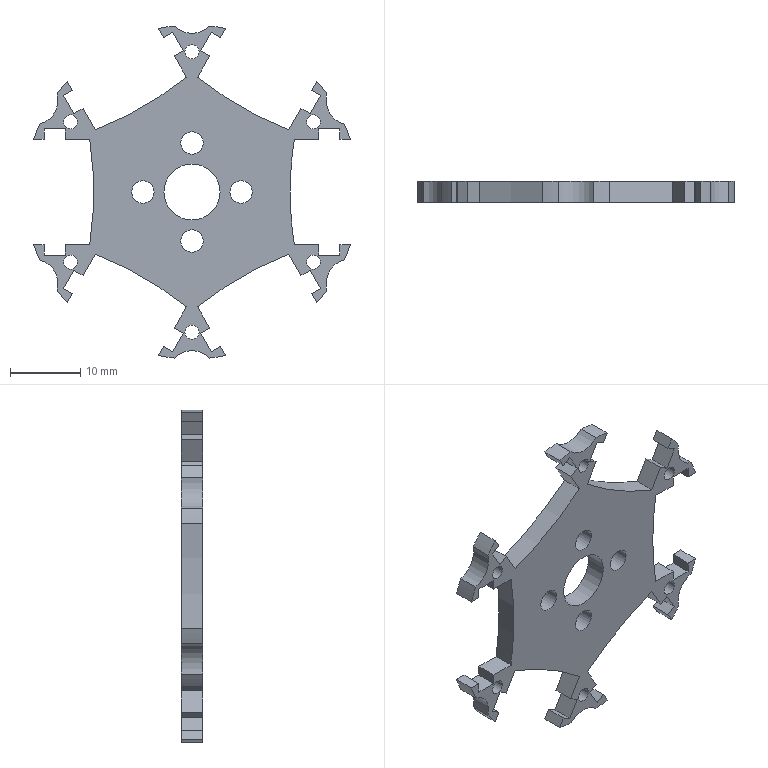Component | SolidWorks | Half-1_MiddleChip-1 | 1 solid | 111 faces | box 45.17 x 3 x 47.34 mm | volume 2314 mm3 | plane 62 | cylinder 49 | commonest cylinder face diameters 2 x12 47.6 x12 3.2 x8 7 x8 96.351 x7 8 x2 | material 1060 Alloy
build123d program:
from build123d import *

# Parameters (mm, degrees)
SKETCH1_R           = 1
SKETCH1_R_2         = 1.6
SKETCH1_R_3         = 4
BOSS_EXTRUDE1_DEPTH = 3


with BuildPart() as part:
    # Sketch1 → Boss-Extrude1 (new body)
    with BuildSketch(Plane.XY):
        with BuildLine():
            ThreePointArc((30.834, 20.027), (24.046, 23.268), (17.844, 27.527))
            Line((17.844, 27.527), (19.594, 30.558))
            Line((19.594, 30.558), (18.295, 31.308))
            Line((18.295, 31.308), (19.795, 33.906))
            Line((19.795, 33.906), (21.094, 33.156))
            Line((21.094, 33.156), (21.844, 34.455))
            ThreePointArc((21.844, 34.455), (20.699, 34.662), (19.546, 34.812))
            ThreePointArc((19.546, 34.812), (17.046, 33.762), (14.546, 34.812))
            ThreePointArc((14.546, 34.812), (13.392, 34.662), (12.247, 34.455))
            Line((12.247, 34.455), (12.997, 33.156))
            Line((12.997, 33.156), (14.296, 33.906))
            Line((14.296, 33.906), (15.796, 31.308))
            Line((15.796, 31.308), (14.497, 30.558))
            Line((14.497, 30.558), (16.247, 27.527))
            ThreePointArc((16.247, 27.527), (10.046, 23.268), (3.257, 20.027))
            Line((3.257, 20.027), (1.507, 23.058))
            Line((1.507, 23.058), (0.2076, 22.308))
            Line((0.2076, 22.308), (-1.292, 24.906))
            Line((-1.292, 24.906), (0.006637, 25.656))
            Line((0.006637, 25.656), (-0.7434, 26.955))
            ThreePointArc((-0.7434, 26.955), (-1.495, 26.067), (-2.202, 25.143))
            ThreePointArc((-2.202, 25.143), (-2.542, 22.453), (-4.702, 20.813))
            ThreePointArc((-4.702, 20.813), (-5.148, 19.738), (-5.542, 18.644))
            Line((-5.542, 18.644), (-4.042, 18.644))
            Line((-4.042, 18.644), (-4.042, 20.144))
            Line((-4.042, 20.144), (-1.042, 20.144))
            Line((-1.042, 20.144), (-1.042, 18.644))
            Line((-1.042, 18.644), (2.458, 18.644))
            ThreePointArc((2.458, 18.644), (3.046, 11.144), (2.458, 3.644))
            Line((2.458, 3.644), (-1.042, 3.644))
            Line((-1.042, 3.644), (-1.042, 2.144))
            Line((-1.042, 2.144), (-4.042, 2.144))
            Line((-4.042, 2.144), (-4.042, 3.644))
            Line((-4.042, 3.644), (-5.542, 3.644))
            ThreePointArc((-5.542, 3.644), (-5.148, 2.549), (-4.702, 1.475))
            ThreePointArc((-4.702, 1.475), (-2.542, -0.1652), (-2.202, -2.856))
            ThreePointArc((-2.202, -2.856), (-1.495, -3.779), (-0.7434, -4.668))
            Line((-0.7434, -4.668), (0.006637, -3.369))
            Line((0.006637, -3.369), (-1.292, -2.619))
            Line((-1.292, -2.619), (0.2076, -0.02046))
            Line((0.2076, -0.02046), (1.507, -0.7705))
            Line((1.507, -0.7705), (3.257, 2.261))
            ThreePointArc((3.257, 2.261), (10.046, -0.9807), (16.247, -5.239))
            Line((16.247, -5.239), (14.497, -8.27))
            Line((14.497, -8.27), (15.796, -9.02))
            Line((15.796, -9.02), (14.296, -11.619))
            Line((14.296, -11.619), (12.997, -10.869))
            Line((12.997, -10.869), (12.247, -12.168))
            ThreePointArc((12.247, -12.168), (13.392, -12.374), (14.546, -12.525))
            ThreePointArc((14.546, -12.525), (17.046, -11.474), (19.546, -12.525))
            ThreePointArc((19.546, -12.525), (20.699, -12.374), (21.844, -12.168))
            Line((21.844, -12.168), (21.094, -10.869))
            Line((21.094, -10.869), (19.795, -11.619))
            Line((19.795, -11.619), (18.295, -9.02))
            Line((18.295, -9.02), (19.594, -8.27))
            Line((19.594, -8.27), (17.844, -5.239))
            ThreePointArc((17.844, -5.239), (24.046, -0.9807), (30.834, 2.261))
            Line((30.834, 2.261), (32.584, -0.7705))
            Line((32.584, -0.7705), (33.883, -0.02046))
            Line((33.883, -0.02046), (35.383, -2.619))
            Line((35.383, -2.619), (34.084, -3.369))
            Line((34.084, -3.369), (34.834, -4.668))
            ThreePointArc((34.834, -4.668), (35.586, -3.779), (36.293, -2.856))
            ThreePointArc((36.293, -2.856), (36.633, -0.1652), (38.793, 1.475))
            ThreePointArc((38.793, 1.475), (39.239, 2.549), (39.633, 3.644))
            Line((39.633, 3.644), (38.133, 3.644))
            Line((38.133, 3.644), (38.133, 2.144))
            Line((38.133, 2.144), (35.133, 2.144))
            Line((35.133, 2.144), (35.133, 3.644))
            Line((35.133, 3.644), (31.633, 3.644))
            ThreePointArc((31.633, 3.644), (31.046, 11.144), (31.633, 18.644))
            Line((31.633, 18.644), (35.133, 18.644))
            Line((35.133, 18.644), (35.133, 20.144))
            Line((35.133, 20.144), (38.133, 20.144))
            Line((38.133, 20.144), (38.133, 18.644))
            Line((38.133, 18.644), (39.633, 18.644))
            ThreePointArc((39.633, 18.644), (39.239, 19.738), (38.793, 20.813))
            ThreePointArc((38.793, 20.813), (36.633, 22.453), (36.293, 25.143))
            ThreePointArc((36.293, 25.143), (35.586, 26.067), (34.834, 26.955))
            Line((34.834, 26.955), (34.084, 25.656))
            Line((34.084, 25.656), (35.383, 24.906))
            Line((35.383, 24.906), (33.883, 22.308))
            Line((33.883, 22.308), (32.584, 23.058))
            Line((32.584, 23.058), (30.834, 20.027))
        make_face()
        with Locations((-0.275, 1.144)):
            Circle(SKETCH1_R, mode=Mode.SUBTRACT)
        with Locations((17.046, -8.856)):
            Circle(SKETCH1_R, mode=Mode.SUBTRACT)
        with Locations((17.046, 4.144)):
            Circle(SKETCH1_R_2, mode=Mode.SUBTRACT)
        with Locations((34.366, 1.144)):
            Circle(SKETCH1_R, mode=Mode.SUBTRACT)
        with Locations((-0.275, 21.144)):
            Circle(SKETCH1_R, mode=Mode.SUBTRACT)
        with Locations((10.046, 11.144)):
            Circle(SKETCH1_R_2, mode=Mode.SUBTRACT)
        with Locations((17.046, 11.144)):
            Circle(SKETCH1_R_3, mode=Mode.SUBTRACT)
        with BuildLine():
            ThreePointArc((25.642, 11.033), (25.431, 10.344), (24.94, 9.817))
            ThreePointArc((24.94, 9.817), (22.633, 11.895), (25.646, 11.144))
            ThreePointArc((25.646, 11.144), (25.645, 11.088), (25.642, 11.033))
        make_face(mode=Mode.SUBTRACT)
        with Locations((17.046, 18.144)):
            Circle(SKETCH1_R_2, mode=Mode.SUBTRACT)
        with Locations((34.366, 21.144)):
            Circle(SKETCH1_R, mode=Mode.SUBTRACT)
        with Locations((17.046, 31.144)):
            Circle(SKETCH1_R, mode=Mode.SUBTRACT)
    extrude(amount=BOSS_EXTRUDE1_DEPTH)


solid = part.part

# Placed as in the assembly
solid = solid.moved(Location((-16.727, -0.6003, 25.856), (90, 0, 0)))